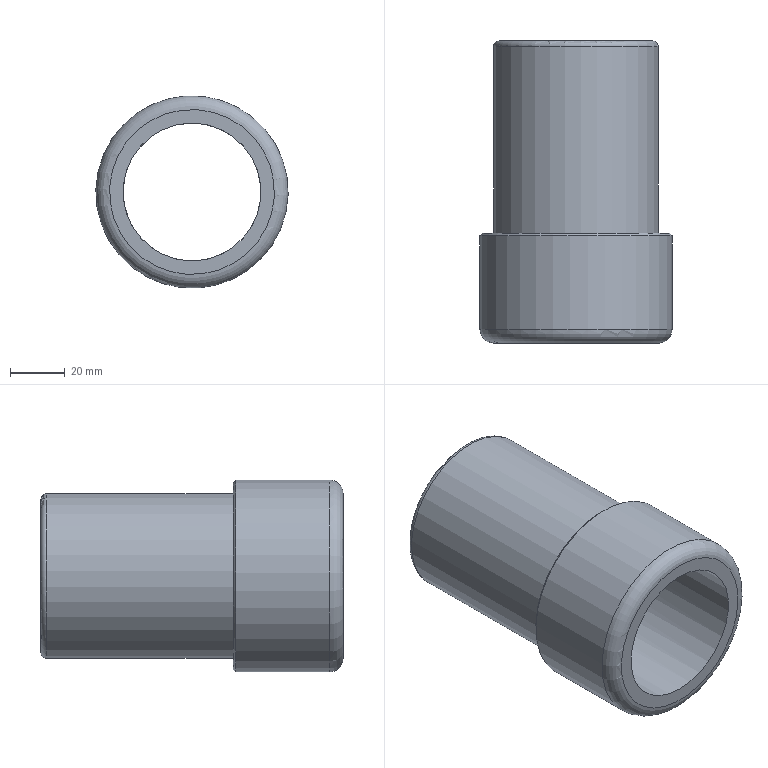Component | NX | BUSH | 1 solid | 10 faces | box 70 x 110 x 70 mm | volume 133028 mm3 | plane 3 | cylinder 3 | torus 3 | cone 1 | commonest cylinder face diameters 70 x1 60 x1 50.15 x1
STEP:
#1=CARTESIAN_POINT('',(0.,0.,0.));
#2=DIRECTION('',(0.,0.,1.));
#3=DIRECTION('',(1.,0.,0.));
#4=AXIS2_PLACEMENT_3D('',#1,#2,#3);
#5=CARTESIAN_POINT('',(-145.981,270.,-222.846));
#6=VERTEX_POINT('',#5);
#7=CARTESIAN_POINT('',(-120.,270.,-207.846));
#8=DIRECTION('',(-0.,-1.,-0.));
#9=DIRECTION('',(-0.866,0.,-0.5));
#10=AXIS2_PLACEMENT_3D('',#7,#8,#9);
#11=CIRCLE('',#10,30.);
#12=CARTESIAN_POINT('',(-120.,270.,-207.846));
#13=DIRECTION('',(0.,1.,0.));
#14=DIRECTION('',(-0.866,0.,-0.5));
#15=AXIS2_PLACEMENT_3D('',#12,#13,#14);
#16=PLANE('',#15);
#17=CARTESIAN_POINT('',(30.,0.));
#18=CARTESIAN_POINT('',(30.,-51.962));
#19=CARTESIAN_POINT('',(-15.,-25.981));
#20=CARTESIAN_POINT('',(-60.,-0.));
#21=CARTESIAN_POINT('',(-15.,25.981));
#22=CARTESIAN_POINT('',(30.,51.962));
#23=CARTESIAN_POINT('',(30.,0.));
#24=(BOUNDED_CURVE()B_SPLINE_CURVE(2,(#17,#18,#19,#20,#21,#22,#23),.UNSPECIFIED.,.T.,.F.)B_SPLINE_CURVE_WITH_KNOTS((1,2,2,2,2,1),(-2.094,0.,2.094,4.189,6.283,8.378),.UNSPECIFIED.)CURVE()GEOMETRIC_REPRESENTATION_ITEM()RATIONAL_B_SPLINE_CURVE((1.,0.5,1.,0.5,1.,0.5,1.))REPRESENTATION_ITEM(''));
#25=(GEOMETRIC_REPRESENTATION_CONTEXT(2)PARAMETRIC_REPRESENTATION_CONTEXT()REPRESENTATION_CONTEXT('',''));
#26=DEFINITIONAL_REPRESENTATION('',(#24),#25);
#27=PCURVE('',#16,#26);
#28=CARTESIAN_POINT('',(-120.,275.,-207.846));
#29=DIRECTION('',(0.,1.,0.));
#30=DIRECTION('',(-0.866,0.,-0.5));
#31=AXIS2_PLACEMENT_3D('',#28,#29,#30);
#32=TOROIDAL_SURFACE('',#31,30.,5.);
#33=CARTESIAN_POINT('',(6.283,4.712));
#34=DIRECTION('',(-1.,0.));
#35=VECTOR('',#34,1.);
#36=LINE('',#33,#35);
#37=(GEOMETRIC_REPRESENTATION_CONTEXT(2)PARAMETRIC_REPRESENTATION_CONTEXT()REPRESENTATION_CONTEXT('',''));
#38=DEFINITIONAL_REPRESENTATION('',(#36),#37);
#39=PCURVE('',#32,#38);
#40=SURFACE_CURVE('',#11,(#27,#39),.PCURVE_S1.);
#41=EDGE_CURVE('',#6,#6,#40,.T.);
#42=ORIENTED_EDGE('',*,*,#41,.T.);
#43=EDGE_LOOP('',(#42));
#44=FACE_BOUND('',#43,.T.);
#45=CARTESIAN_POINT('',(-141.716,270.,-220.384));
#46=VERTEX_POINT('',#45);
#47=CARTESIAN_POINT('',(-98.284,270.,-195.309));
#48=VERTEX_POINT('',#47);
#49=CARTESIAN_POINT('',(-120.,270.,-207.846));
#50=DIRECTION('',(0.,1.,0.));
#51=DIRECTION('',(-0.866,0.,-0.5));
#52=AXIS2_PLACEMENT_3D('',#49,#50,#51);
#53=CIRCLE('',#52,25.075);
#54=CARTESIAN_POINT('',(0.,0.));
#55=DIRECTION('',(1.,0.));
#56=AXIS2_PLACEMENT_2D('',#54,#55);
#57=CIRCLE('',#56,25.075);
#58=(GEOMETRIC_REPRESENTATION_CONTEXT(2)PARAMETRIC_REPRESENTATION_CONTEXT()REPRESENTATION_CONTEXT('',''));
#59=DEFINITIONAL_REPRESENTATION('',(#57),#58);
#60=PCURVE('',#16,#59);
#61=CARTESIAN_POINT('',(-120.,380.,-207.846));
#62=DIRECTION('',(-0.,-1.,-0.));
#63=DIRECTION('',(0.866,-0.,0.5));
#64=AXIS2_PLACEMENT_3D('',#61,#62,#63);
#65=CYLINDRICAL_SURFACE('',#64,25.075);
#66=CARTESIAN_POINT('',(3.142,110.));
#67=DIRECTION('',(-1.,0.));
#68=VECTOR('',#67,1.);
#69=LINE('',#66,#68);
#70=(GEOMETRIC_REPRESENTATION_CONTEXT(2)PARAMETRIC_REPRESENTATION_CONTEXT()REPRESENTATION_CONTEXT('',''));
#71=DEFINITIONAL_REPRESENTATION('',(#69),#70);
#72=PCURVE('',#65,#71);
#73=SURFACE_CURVE('',#53,(#60,#72),.PCURVE_S1.);
#74=EDGE_CURVE('',#46,#48,#73,.T.);
#75=ORIENTED_EDGE('',*,*,#74,.T.);
#76=CARTESIAN_POINT('',(-120.,270.,-207.846));
#77=DIRECTION('',(0.,1.,0.));
#78=DIRECTION('',(-0.866,0.,-0.5));
#79=AXIS2_PLACEMENT_3D('',#76,#77,#78);
#80=CIRCLE('',#79,25.075);
#81=CARTESIAN_POINT('',(0.,0.));
#82=DIRECTION('',(1.,0.));
#83=AXIS2_PLACEMENT_2D('',#81,#82);
#84=CIRCLE('',#83,25.075);
#85=(GEOMETRIC_REPRESENTATION_CONTEXT(2)PARAMETRIC_REPRESENTATION_CONTEXT()REPRESENTATION_CONTEXT('',''));
#86=DEFINITIONAL_REPRESENTATION('',(#84),#85);
#87=PCURVE('',#16,#86);
#88=CARTESIAN_POINT('',(9.425,110.));
#89=DIRECTION('',(-1.,0.));
#90=VECTOR('',#89,1.);
#91=LINE('',#88,#90);
#92=(GEOMETRIC_REPRESENTATION_CONTEXT(2)PARAMETRIC_REPRESENTATION_CONTEXT()REPRESENTATION_CONTEXT('',''));
#93=DEFINITIONAL_REPRESENTATION('',(#91),#92);
#94=PCURVE('',#65,#93);
#95=SURFACE_CURVE('',#80,(#87,#94),.PCURVE_S1.);
#96=EDGE_CURVE('',#48,#46,#95,.T.);
#97=ORIENTED_EDGE('',*,*,#96,.T.);
#98=EDGE_LOOP('',(#75,#97));
#99=FACE_BOUND('',#98,.T.);
#100=ADVANCED_FACE('',(#44,#99),#16,.F.);
#101=CARTESIAN_POINT('',(-89.689,309.,-190.346));
#102=VERTEX_POINT('',#101);
#103=CARTESIAN_POINT('',(-150.311,309.,-225.346));
#104=VERTEX_POINT('',#103);
#105=CARTESIAN_POINT('',(-120.,309.,-207.846));
#106=DIRECTION('',(-0.,-1.,-0.));
#107=DIRECTION('',(0.866,-0.,0.5));
#108=AXIS2_PLACEMENT_3D('',#105,#106,#107);
#109=CIRCLE('',#108,35.);
#110=CARTESIAN_POINT('',(-120.,270.,-207.846));
#111=DIRECTION('',(0.,1.,0.));
#112=DIRECTION('',(-0.866,0.,-0.5));
#113=AXIS2_PLACEMENT_3D('',#110,#111,#112);
#114=CYLINDRICAL_SURFACE('',#113,35.);
#115=CARTESIAN_POINT('',(3.142,39.));
#116=DIRECTION('',(-1.,0.));
#117=VECTOR('',#116,1.);
#118=LINE('',#115,#117);
#119=(GEOMETRIC_REPRESENTATION_CONTEXT(2)PARAMETRIC_REPRESENTATION_CONTEXT()REPRESENTATION_CONTEXT('',''));
#120=DEFINITIONAL_REPRESENTATION('',(#118),#119);
#121=PCURVE('',#114,#120);
#122=CARTESIAN_POINT('',(-120.,310.,-207.846));
#123=DIRECTION('',(-0.,-1.,-0.));
#124=DIRECTION('',(0.866,-0.,0.5));
#125=AXIS2_PLACEMENT_3D('',#122,#123,#124);
#126=CONICAL_SURFACE('',#125,34.,0.7854);
#127=CARTESIAN_POINT('',(0.,1.));
#128=DIRECTION('',(1.,0.));
#129=VECTOR('',#128,1.);
#130=LINE('',#127,#129);
#131=(GEOMETRIC_REPRESENTATION_CONTEXT(2)PARAMETRIC_REPRESENTATION_CONTEXT()REPRESENTATION_CONTEXT('',''));
#132=DEFINITIONAL_REPRESENTATION('',(#130),#131);
#133=PCURVE('',#126,#132);
#134=SURFACE_CURVE('',#109,(#121,#133),.PCURVE_S1.);
#135=EDGE_CURVE('',#102,#104,#134,.T.);
#136=ORIENTED_EDGE('',*,*,#135,.T.);
#137=CARTESIAN_POINT('',(-150.311,275.,-225.346));
#138=VERTEX_POINT('',#137);
#139=CARTESIAN_POINT('',(-150.311,275.,-225.346));
#140=CARTESIAN_POINT('',(-150.311,309.,-225.346));
#141=B_SPLINE_CURVE_WITH_KNOTS('',1,(#139,#140),.UNSPECIFIED.,.F.,.F.,(2,2),(5.,39.),.PIECEWISE_BEZIER_KNOTS.);
#142=CARTESIAN_POINT('',(0.,0.));
#143=DIRECTION('',(0.,1.));
#144=VECTOR('',#143,1.);
#145=LINE('',#142,#144);
#146=(GEOMETRIC_REPRESENTATION_CONTEXT(2)PARAMETRIC_REPRESENTATION_CONTEXT()REPRESENTATION_CONTEXT('',''));
#147=DEFINITIONAL_REPRESENTATION('',(#145),#146);
#148=PCURVE('',#114,#147);
#149=CARTESIAN_POINT('',(6.283,0.));
#150=DIRECTION('',(0.,1.));
#151=VECTOR('',#150,1.);
#152=LINE('',#149,#151);
#153=(GEOMETRIC_REPRESENTATION_CONTEXT(2)PARAMETRIC_REPRESENTATION_CONTEXT()REPRESENTATION_CONTEXT('',''));
#154=DEFINITIONAL_REPRESENTATION('',(#152),#153);
#155=PCURVE('',#114,#154);
#156=SEAM_CURVE('',#141,(#148,#155),.PCURVE_S1.);
#157=EDGE_CURVE('',#138,#104,#156,.T.);
#158=ORIENTED_EDGE('',*,*,#157,.F.);
#159=CARTESIAN_POINT('',(-120.,275.,-207.846));
#160=DIRECTION('',(0.,1.,0.));
#161=DIRECTION('',(-0.866,0.,-0.5));
#162=AXIS2_PLACEMENT_3D('',#159,#160,#161);
#163=CIRCLE('',#162,35.);
#164=CARTESIAN_POINT('',(0.,5.));
#165=DIRECTION('',(1.,0.));
#166=VECTOR('',#165,1.);
#167=LINE('',#164,#166);
#168=(GEOMETRIC_REPRESENTATION_CONTEXT(2)PARAMETRIC_REPRESENTATION_CONTEXT()REPRESENTATION_CONTEXT('',''));
#169=DEFINITIONAL_REPRESENTATION('',(#167),#168);
#170=PCURVE('',#114,#169);
#171=CARTESIAN_POINT('',(0.,6.283));
#172=DIRECTION('',(1.,0.));
#173=VECTOR('',#172,1.);
#174=LINE('',#171,#173);
#175=(GEOMETRIC_REPRESENTATION_CONTEXT(2)PARAMETRIC_REPRESENTATION_CONTEXT()REPRESENTATION_CONTEXT('',''));
#176=DEFINITIONAL_REPRESENTATION('',(#174),#175);
#177=PCURVE('',#32,#176);
#178=SURFACE_CURVE('',#163,(#170,#177),.PCURVE_S1.);
#179=EDGE_CURVE('',#138,#138,#178,.T.);
#180=ORIENTED_EDGE('',*,*,#179,.T.);
#181=ORIENTED_EDGE('',*,*,#157,.T.);
#182=CARTESIAN_POINT('',(-120.,309.,-207.846));
#183=DIRECTION('',(-0.,-1.,-0.));
#184=DIRECTION('',(0.866,-0.,0.5));
#185=AXIS2_PLACEMENT_3D('',#182,#183,#184);
#186=CIRCLE('',#185,35.);
#187=CARTESIAN_POINT('',(9.425,39.));
#188=DIRECTION('',(-1.,0.));
#189=VECTOR('',#188,1.);
#190=LINE('',#187,#189);
#191=(GEOMETRIC_REPRESENTATION_CONTEXT(2)PARAMETRIC_REPRESENTATION_CONTEXT()REPRESENTATION_CONTEXT('',''));
#192=DEFINITIONAL_REPRESENTATION('',(#190),#191);
#193=PCURVE('',#114,#192);
#194=CARTESIAN_POINT('',(0.,1.));
#195=DIRECTION('',(1.,-0.));
#196=VECTOR('',#195,1.);
#197=LINE('',#194,#196);
#198=(GEOMETRIC_REPRESENTATION_CONTEXT(2)PARAMETRIC_REPRESENTATION_CONTEXT()REPRESENTATION_CONTEXT('',''));
#199=DEFINITIONAL_REPRESENTATION('',(#197),#198);
#200=PCURVE('',#126,#199);
#201=SURFACE_CURVE('',#186,(#193,#200),.PCURVE_S1.);
#202=EDGE_CURVE('',#104,#102,#201,.T.);
#203=ORIENTED_EDGE('',*,*,#202,.T.);
#204=EDGE_LOOP('',(#136,#158,#180,#181,#203));
#205=FACE_BOUND('',#204,.T.);
#206=ADVANCED_FACE('',(#205),#114,.T.);
#207=CARTESIAN_POINT('',(-90.555,310.,-190.846));
#208=VERTEX_POINT('',#207);
#209=CARTESIAN_POINT('',(-120.,310.,-207.846));
#210=DIRECTION('',(0.,1.,0.));
#211=DIRECTION('',(0.866,-0.,0.5));
#212=AXIS2_PLACEMENT_3D('',#209,#210,#211);
#213=CIRCLE('',#212,34.);
#214=CARTESIAN_POINT('',(-89.689,310.,-190.346));
#215=DIRECTION('',(-0.,-1.,-0.));
#216=DIRECTION('',(0.866,-0.,0.5));
#217=AXIS2_PLACEMENT_3D('',#214,#215,#216);
#218=PLANE('',#217);
#219=CARTESIAN_POINT('',(-1.,0.));
#220=CARTESIAN_POINT('',(-1.,-58.89));
#221=CARTESIAN_POINT('',(-52.,-29.445));
#222=CARTESIAN_POINT('',(-103.,0.));
#223=CARTESIAN_POINT('',(-52.,29.445));
#224=CARTESIAN_POINT('',(-1.,58.89));
#225=CARTESIAN_POINT('',(-1.,0.));
#226=(BOUNDED_CURVE()B_SPLINE_CURVE(2,(#219,#220,#221,#222,#223,#224,#225),.UNSPECIFIED.,.T.,.F.)B_SPLINE_CURVE_WITH_KNOTS((1,2,2,2,2,1),(-2.094,0.,2.094,4.189,6.283,8.378),.UNSPECIFIED.)CURVE()GEOMETRIC_REPRESENTATION_ITEM()RATIONAL_B_SPLINE_CURVE((1.,0.5,1.,0.5,1.,0.5,1.))REPRESENTATION_ITEM(''));
#227=(GEOMETRIC_REPRESENTATION_CONTEXT(2)PARAMETRIC_REPRESENTATION_CONTEXT()REPRESENTATION_CONTEXT('',''));
#228=DEFINITIONAL_REPRESENTATION('',(#226),#227);
#229=PCURVE('',#218,#228);
#230=CARTESIAN_POINT('',(6.283,-0.));
#231=DIRECTION('',(-1.,0.));
#232=VECTOR('',#231,1.);
#233=LINE('',#230,#232);
#234=(GEOMETRIC_REPRESENTATION_CONTEXT(2)PARAMETRIC_REPRESENTATION_CONTEXT()REPRESENTATION_CONTEXT('',''));
#235=DEFINITIONAL_REPRESENTATION('',(#233),#234);
#236=PCURVE('',#126,#235);
#237=SURFACE_CURVE('',#213,(#229,#236),.PCURVE_S1.);
#238=EDGE_CURVE('',#208,#208,#237,.T.);
#239=ORIENTED_EDGE('',*,*,#238,.T.);
#240=EDGE_LOOP('',(#239));
#241=FACE_BOUND('',#240,.T.);
#242=CARTESIAN_POINT('',(-145.981,310.,-222.846));
#243=VERTEX_POINT('',#242);
#244=CARTESIAN_POINT('',(-120.,310.,-207.846));
#245=DIRECTION('',(0.,1.,0.));
#246=DIRECTION('',(-0.866,0.,-0.5));
#247=AXIS2_PLACEMENT_3D('',#244,#245,#246);
#248=CIRCLE('',#247,30.);
#249=CARTESIAN_POINT('',(-65.,0.));
#250=CARTESIAN_POINT('',(-65.,51.962));
#251=CARTESIAN_POINT('',(-20.,25.981));
#252=CARTESIAN_POINT('',(25.,0.));
#253=CARTESIAN_POINT('',(-20.,-25.981));
#254=CARTESIAN_POINT('',(-65.,-51.962));
#255=CARTESIAN_POINT('',(-65.,0.));
#256=(BOUNDED_CURVE()B_SPLINE_CURVE(2,(#249,#250,#251,#252,#253,#254,#255),.UNSPECIFIED.,.T.,.F.)B_SPLINE_CURVE_WITH_KNOTS((1,2,2,2,2,1),(-2.094,0.,2.094,4.189,6.283,8.378),.UNSPECIFIED.)CURVE()GEOMETRIC_REPRESENTATION_ITEM()RATIONAL_B_SPLINE_CURVE((1.,0.5,1.,0.5,1.,0.5,1.))REPRESENTATION_ITEM(''));
#257=(GEOMETRIC_REPRESENTATION_CONTEXT(2)PARAMETRIC_REPRESENTATION_CONTEXT()REPRESENTATION_CONTEXT('',''));
#258=DEFINITIONAL_REPRESENTATION('',(#256),#257);
#259=PCURVE('',#218,#258);
#260=CARTESIAN_POINT('',(-120.,270.,-207.846));
#261=DIRECTION('',(0.,1.,0.));
#262=DIRECTION('',(-0.866,0.,-0.5));
#263=AXIS2_PLACEMENT_3D('',#260,#261,#262);
#264=CYLINDRICAL_SURFACE('',#263,30.);
#265=CARTESIAN_POINT('',(0.,40.));
#266=DIRECTION('',(1.,0.));
#267=VECTOR('',#266,1.);
#268=LINE('',#265,#267);
#269=(GEOMETRIC_REPRESENTATION_CONTEXT(2)PARAMETRIC_REPRESENTATION_CONTEXT()REPRESENTATION_CONTEXT('',''));
#270=DEFINITIONAL_REPRESENTATION('',(#268),#269);
#271=PCURVE('',#264,#270);
#272=SURFACE_CURVE('',#248,(#259,#271),.PCURVE_S1.);
#273=EDGE_CURVE('',#243,#243,#272,.T.);
#274=ORIENTED_EDGE('',*,*,#273,.F.);
#275=EDGE_LOOP('',(#274));
#276=FACE_BOUND('',#275,.T.);
#277=ADVANCED_FACE('',(#241,#276),#218,.F.);
#278=CARTESIAN_POINT('',(-94.019,378.,-192.846));
#279=VERTEX_POINT('',#278);
#280=CARTESIAN_POINT('',(-145.981,378.,-222.846));
#281=VERTEX_POINT('',#280);
#282=CARTESIAN_POINT('',(-120.,378.,-207.846));
#283=DIRECTION('',(-0.,-1.,-0.));
#284=DIRECTION('',(0.866,-0.,0.5));
#285=AXIS2_PLACEMENT_3D('',#282,#283,#284);
#286=CIRCLE('',#285,30.);
#287=CARTESIAN_POINT('',(3.142,108.));
#288=DIRECTION('',(-1.,0.));
#289=VECTOR('',#288,1.);
#290=LINE('',#287,#289);
#291=(GEOMETRIC_REPRESENTATION_CONTEXT(2)PARAMETRIC_REPRESENTATION_CONTEXT()REPRESENTATION_CONTEXT('',''));
#292=DEFINITIONAL_REPRESENTATION('',(#290),#291);
#293=PCURVE('',#264,#292);
#294=CARTESIAN_POINT('',(-120.,378.,-207.846));
#295=DIRECTION('',(-0.,-1.,-0.));
#296=DIRECTION('',(0.866,-0.,0.5));
#297=AXIS2_PLACEMENT_3D('',#294,#295,#296);
#298=TOROIDAL_SURFACE('',#297,28.,2.);
#299=CARTESIAN_POINT('',(0.,6.283));
#300=DIRECTION('',(1.,0.));
#301=VECTOR('',#300,1.);
#302=LINE('',#299,#301);
#303=(GEOMETRIC_REPRESENTATION_CONTEXT(2)PARAMETRIC_REPRESENTATION_CONTEXT()REPRESENTATION_CONTEXT('',''));
#304=DEFINITIONAL_REPRESENTATION('',(#302),#303);
#305=PCURVE('',#298,#304);
#306=SURFACE_CURVE('',#286,(#293,#305),.PCURVE_S1.);
#307=EDGE_CURVE('',#279,#281,#306,.T.);
#308=ORIENTED_EDGE('',*,*,#307,.T.);
#309=CARTESIAN_POINT('',(-145.981,310.,-222.846));
#310=CARTESIAN_POINT('',(-145.981,378.,-222.846));
#311=B_SPLINE_CURVE_WITH_KNOTS('',1,(#309,#310),.UNSPECIFIED.,.F.,.F.,(2,2),(40.,108.),.PIECEWISE_BEZIER_KNOTS.);
#312=CARTESIAN_POINT('',(0.,0.));
#313=DIRECTION('',(0.,1.));
#314=VECTOR('',#313,1.);
#315=LINE('',#312,#314);
#316=(GEOMETRIC_REPRESENTATION_CONTEXT(2)PARAMETRIC_REPRESENTATION_CONTEXT()REPRESENTATION_CONTEXT('',''));
#317=DEFINITIONAL_REPRESENTATION('',(#315),#316);
#318=PCURVE('',#264,#317);
#319=CARTESIAN_POINT('',(6.283,0.));
#320=DIRECTION('',(0.,1.));
#321=VECTOR('',#320,1.);
#322=LINE('',#319,#321);
#323=(GEOMETRIC_REPRESENTATION_CONTEXT(2)PARAMETRIC_REPRESENTATION_CONTEXT()REPRESENTATION_CONTEXT('',''));
#324=DEFINITIONAL_REPRESENTATION('',(#322),#323);
#325=PCURVE('',#264,#324);
#326=SEAM_CURVE('',#311,(#318,#325),.PCURVE_S1.);
#327=EDGE_CURVE('',#243,#281,#326,.T.);
#328=ORIENTED_EDGE('',*,*,#327,.F.);
#329=ORIENTED_EDGE('',*,*,#273,.T.);
#330=ORIENTED_EDGE('',*,*,#327,.T.);
#331=CARTESIAN_POINT('',(-120.,378.,-207.846));
#332=DIRECTION('',(-0.,-1.,-0.));
#333=DIRECTION('',(0.866,-0.,0.5));
#334=AXIS2_PLACEMENT_3D('',#331,#332,#333);
#335=CIRCLE('',#334,30.);
#336=CARTESIAN_POINT('',(9.425,108.));
#337=DIRECTION('',(-1.,0.));
#338=VECTOR('',#337,1.);
#339=LINE('',#336,#338);
#340=(GEOMETRIC_REPRESENTATION_CONTEXT(2)PARAMETRIC_REPRESENTATION_CONTEXT()REPRESENTATION_CONTEXT('',''));
#341=DEFINITIONAL_REPRESENTATION('',(#339),#340);
#342=PCURVE('',#264,#341);
#343=CARTESIAN_POINT('',(0.,6.283));
#344=DIRECTION('',(1.,0.));
#345=VECTOR('',#344,1.);
#346=LINE('',#343,#345);
#347=(GEOMETRIC_REPRESENTATION_CONTEXT(2)PARAMETRIC_REPRESENTATION_CONTEXT()REPRESENTATION_CONTEXT('',''));
#348=DEFINITIONAL_REPRESENTATION('',(#346),#347);
#349=PCURVE('',#298,#348);
#350=SURFACE_CURVE('',#335,(#342,#349),.PCURVE_S1.);
#351=EDGE_CURVE('',#281,#279,#350,.T.);
#352=ORIENTED_EDGE('',*,*,#351,.T.);
#353=EDGE_LOOP('',(#308,#328,#329,#330,#352));
#354=FACE_BOUND('',#353,.T.);
#355=ADVANCED_FACE('',(#354),#264,.T.);
#356=CARTESIAN_POINT('',(-96.552,380.,-194.309));
#357=VERTEX_POINT('',#356);
#358=CARTESIAN_POINT('',(-120.,380.,-207.846));
#359=DIRECTION('',(-0.,-1.,-0.));
#360=DIRECTION('',(0.866,-0.,0.5));
#361=AXIS2_PLACEMENT_3D('',#358,#359,#360);
#362=CIRCLE('',#361,27.075);
#363=CARTESIAN_POINT('',(-94.019,380.,-192.846));
#364=DIRECTION('',(-0.,-1.,-0.));
#365=DIRECTION('',(0.866,-0.,0.5));
#366=AXIS2_PLACEMENT_3D('',#363,#364,#365);
#367=PLANE('',#366);
#368=CARTESIAN_POINT('',(-30.,0.));
#369=DIRECTION('',(1.,0.));
#370=AXIS2_PLACEMENT_2D('',#368,#369);
#371=CIRCLE('',#370,27.075);
#372=(GEOMETRIC_REPRESENTATION_CONTEXT(2)PARAMETRIC_REPRESENTATION_CONTEXT()REPRESENTATION_CONTEXT('',''));
#373=DEFINITIONAL_REPRESENTATION('',(#371),#372);
#374=PCURVE('',#367,#373);
#375=CARTESIAN_POINT('',(-120.,378.,-207.846));
#376=DIRECTION('',(-0.,-1.,-0.));
#377=DIRECTION('',(0.866,-0.,0.5));
#378=AXIS2_PLACEMENT_3D('',#375,#376,#377);
#379=TOROIDAL_SURFACE('',#378,27.075,2.);
#380=CARTESIAN_POINT('',(0.,4.712));
#381=DIRECTION('',(1.,0.));
#382=VECTOR('',#381,1.);
#383=LINE('',#380,#382);
#384=(GEOMETRIC_REPRESENTATION_CONTEXT(2)PARAMETRIC_REPRESENTATION_CONTEXT()REPRESENTATION_CONTEXT('',''));
#385=DEFINITIONAL_REPRESENTATION('',(#383),#384);
#386=PCURVE('',#379,#385);
#387=SURFACE_CURVE('',#362,(#374,#386),.PCURVE_S1.);
#388=EDGE_CURVE('',#357,#357,#387,.T.);
#389=ORIENTED_EDGE('',*,*,#388,.T.);
#390=EDGE_LOOP('',(#389));
#391=FACE_BOUND('',#390,.T.);
#392=CARTESIAN_POINT('',(-95.751,380.,-193.846));
#393=VERTEX_POINT('',#392);
#394=CARTESIAN_POINT('',(-120.,380.,-207.846));
#395=DIRECTION('',(0.,1.,0.));
#396=DIRECTION('',(0.866,-0.,0.5));
#397=AXIS2_PLACEMENT_3D('',#394,#395,#396);
#398=CIRCLE('',#397,28.);
#399=CARTESIAN_POINT('',(-2.,0.));
#400=CARTESIAN_POINT('',(-2.,-48.497));
#401=CARTESIAN_POINT('',(-44.,-24.249));
#402=CARTESIAN_POINT('',(-86.,0.));
#403=CARTESIAN_POINT('',(-44.,24.249));
#404=CARTESIAN_POINT('',(-2.,48.497));
#405=CARTESIAN_POINT('',(-2.,0.));
#406=(BOUNDED_CURVE()B_SPLINE_CURVE(2,(#399,#400,#401,#402,#403,#404,#405),.UNSPECIFIED.,.T.,.F.)B_SPLINE_CURVE_WITH_KNOTS((1,2,2,2,2,1),(-2.094,0.,2.094,4.189,6.283,8.378),.UNSPECIFIED.)CURVE()GEOMETRIC_REPRESENTATION_ITEM()RATIONAL_B_SPLINE_CURVE((1.,0.5,1.,0.5,1.,0.5,1.))REPRESENTATION_ITEM(''));
#407=(GEOMETRIC_REPRESENTATION_CONTEXT(2)PARAMETRIC_REPRESENTATION_CONTEXT()REPRESENTATION_CONTEXT('',''));
#408=DEFINITIONAL_REPRESENTATION('',(#406),#407);
#409=PCURVE('',#367,#408);
#410=CARTESIAN_POINT('',(6.283,4.712));
#411=DIRECTION('',(-1.,0.));
#412=VECTOR('',#411,1.);
#413=LINE('',#410,#412);
#414=(GEOMETRIC_REPRESENTATION_CONTEXT(2)PARAMETRIC_REPRESENTATION_CONTEXT()REPRESENTATION_CONTEXT('',''));
#415=DEFINITIONAL_REPRESENTATION('',(#413),#414);
#416=PCURVE('',#298,#415);
#417=SURFACE_CURVE('',#398,(#409,#416),.PCURVE_S1.);
#418=EDGE_CURVE('',#393,#393,#417,.T.);
#419=ORIENTED_EDGE('',*,*,#418,.T.);
#420=EDGE_LOOP('',(#419));
#421=FACE_BOUND('',#420,.T.);
#422=ADVANCED_FACE('',(#391,#421),#367,.F.);
#423=CARTESIAN_POINT('',(-98.284,378.,-195.309));
#424=VERTEX_POINT('',#423);
#425=CARTESIAN_POINT('',(-120.,378.,-207.846));
#426=DIRECTION('',(0.,1.,0.));
#427=DIRECTION('',(0.866,-0.,0.5));
#428=AXIS2_PLACEMENT_3D('',#425,#426,#427);
#429=CIRCLE('',#428,25.075);
#430=CARTESIAN_POINT('',(6.283,2.));
#431=DIRECTION('',(-1.,0.));
#432=VECTOR('',#431,1.);
#433=LINE('',#430,#432);
#434=(GEOMETRIC_REPRESENTATION_CONTEXT(2)PARAMETRIC_REPRESENTATION_CONTEXT()REPRESENTATION_CONTEXT('',''));
#435=DEFINITIONAL_REPRESENTATION('',(#433),#434);
#436=PCURVE('',#65,#435);
#437=CARTESIAN_POINT('',(6.283,3.142));
#438=DIRECTION('',(-1.,0.));
#439=VECTOR('',#438,1.);
#440=LINE('',#437,#439);
#441=(GEOMETRIC_REPRESENTATION_CONTEXT(2)PARAMETRIC_REPRESENTATION_CONTEXT()REPRESENTATION_CONTEXT('',''));
#442=DEFINITIONAL_REPRESENTATION('',(#440),#441);
#443=PCURVE('',#379,#442);
#444=SURFACE_CURVE('',#429,(#436,#443),.PCURVE_S1.);
#445=EDGE_CURVE('',#424,#424,#444,.T.);
#446=ORIENTED_EDGE('',*,*,#445,.F.);
#447=CARTESIAN_POINT('',(-98.284,378.,-195.309));
#448=CARTESIAN_POINT('',(-98.284,270.,-195.309));
#449=B_SPLINE_CURVE_WITH_KNOTS('',1,(#447,#448),.UNSPECIFIED.,.F.,.F.,(2,2),(2.,110.),.PIECEWISE_BEZIER_KNOTS.);
#450=CARTESIAN_POINT('',(6.283,0.));
#451=DIRECTION('',(0.,1.));
#452=VECTOR('',#451,1.);
#453=LINE('',#450,#452);
#454=(GEOMETRIC_REPRESENTATION_CONTEXT(2)PARAMETRIC_REPRESENTATION_CONTEXT()REPRESENTATION_CONTEXT('',''));
#455=DEFINITIONAL_REPRESENTATION('',(#453),#454);
#456=PCURVE('',#65,#455);
#457=CARTESIAN_POINT('',(0.,0.));
#458=DIRECTION('',(0.,1.));
#459=VECTOR('',#458,1.);
#460=LINE('',#457,#459);
#461=(GEOMETRIC_REPRESENTATION_CONTEXT(2)PARAMETRIC_REPRESENTATION_CONTEXT()REPRESENTATION_CONTEXT('',''));
#462=DEFINITIONAL_REPRESENTATION('',(#460),#461);
#463=PCURVE('',#65,#462);
#464=SEAM_CURVE('',#449,(#456,#463),.PCURVE_S1.);
#465=EDGE_CURVE('',#424,#48,#464,.T.);
#466=ORIENTED_EDGE('',*,*,#465,.T.);
#467=ORIENTED_EDGE('',*,*,#96,.T.);
#468=ORIENTED_EDGE('',*,*,#74,.T.);
#469=ORIENTED_EDGE('',*,*,#465,.F.);
#470=EDGE_LOOP('',(#446,#466,#467,#468,#469));
#471=FACE_BOUND('',#470,.F.);
#472=ADVANCED_FACE('',(#471),#65,.F.);
#473=ORIENTED_EDGE('',*,*,#41,.F.);
#474=CARTESIAN_POINT('',(-145.981,270.,-222.846));
#475=CARTESIAN_POINT('',(-147.138,270.,-223.514));
#476=CARTESIAN_POINT('',(-148.266,270.425,-224.165));
#477=CARTESIAN_POINT('',(-149.237,271.24,-224.726));
#478=CARTESIAN_POINT('',(-149.943,272.361,-225.134));
#479=CARTESIAN_POINT('',(-150.311,273.663,-225.346));
#480=CARTESIAN_POINT('',(-150.311,275.,-225.346));
#481=(BOUNDED_CURVE()B_SPLINE_CURVE(6,(#474,#475,#476,#477,#478,#479,#480),.UNSPECIFIED.,.F.,.F.)B_SPLINE_CURVE_WITH_KNOTS((7,7),(4.712,6.283),.PIECEWISE_BEZIER_KNOTS.)CURVE()GEOMETRIC_REPRESENTATION_ITEM()RATIONAL_B_SPLINE_CURVE((1.031,1.01,0.9979,0.994,0.9979,1.01,1.031))REPRESENTATION_ITEM(''));
#482=CARTESIAN_POINT('',(6.283,0.));
#483=DIRECTION('',(0.,1.));
#484=VECTOR('',#483,1.);
#485=LINE('',#482,#484);
#486=(GEOMETRIC_REPRESENTATION_CONTEXT(2)PARAMETRIC_REPRESENTATION_CONTEXT()REPRESENTATION_CONTEXT('',''));
#487=DEFINITIONAL_REPRESENTATION('',(#485),#486);
#488=PCURVE('',#32,#487);
#489=CARTESIAN_POINT('',(0.,0.));
#490=DIRECTION('',(0.,1.));
#491=VECTOR('',#490,1.);
#492=LINE('',#489,#491);
#493=(GEOMETRIC_REPRESENTATION_CONTEXT(2)PARAMETRIC_REPRESENTATION_CONTEXT()REPRESENTATION_CONTEXT('',''));
#494=DEFINITIONAL_REPRESENTATION('',(#492),#493);
#495=PCURVE('',#32,#494);
#496=SEAM_CURVE('',#481,(#488,#495),.PCURVE_S1.);
#497=EDGE_CURVE('',#6,#138,#496,.T.);
#498=ORIENTED_EDGE('',*,*,#497,.T.);
#499=ORIENTED_EDGE('',*,*,#179,.F.);
#500=ORIENTED_EDGE('',*,*,#497,.F.);
#501=EDGE_LOOP('',(#473,#498,#499,#500));
#502=FACE_BOUND('',#501,.T.);
#503=ADVANCED_FACE('',(#502),#32,.T.);
#504=ORIENTED_EDGE('',*,*,#445,.F.);
#505=CARTESIAN_POINT('',(-98.284,378.,-195.309));
#506=CARTESIAN_POINT('',(-98.284,378.535,-195.309));
#507=CARTESIAN_POINT('',(-98.137,379.055,-195.224));
#508=CARTESIAN_POINT('',(-97.855,379.504,-195.061));
#509=CARTESIAN_POINT('',(-97.466,379.83,-194.836));
#510=CARTESIAN_POINT('',(-97.015,380.,-194.576));
#511=CARTESIAN_POINT('',(-96.552,380.,-194.309));
#512=(BOUNDED_CURVE()B_SPLINE_CURVE(6,(#505,#506,#507,#508,#509,#510,#511),.UNSPECIFIED.,.F.,.F.)B_SPLINE_CURVE_WITH_KNOTS((7,7),(3.142,4.712),.PIECEWISE_BEZIER_KNOTS.)CURVE()GEOMETRIC_REPRESENTATION_ITEM()RATIONAL_B_SPLINE_CURVE((1.031,1.01,0.9979,0.994,0.9979,1.01,1.031))REPRESENTATION_ITEM(''));
#513=CARTESIAN_POINT('',(6.283,0.));
#514=DIRECTION('',(0.,1.));
#515=VECTOR('',#514,1.);
#516=LINE('',#513,#515);
#517=(GEOMETRIC_REPRESENTATION_CONTEXT(2)PARAMETRIC_REPRESENTATION_CONTEXT()REPRESENTATION_CONTEXT('',''));
#518=DEFINITIONAL_REPRESENTATION('',(#516),#517);
#519=PCURVE('',#379,#518);
#520=CARTESIAN_POINT('',(0.,0.));
#521=DIRECTION('',(0.,1.));
#522=VECTOR('',#521,1.);
#523=LINE('',#520,#522);
#524=(GEOMETRIC_REPRESENTATION_CONTEXT(2)PARAMETRIC_REPRESENTATION_CONTEXT()REPRESENTATION_CONTEXT('',''));
#525=DEFINITIONAL_REPRESENTATION('',(#523),#524);
#526=PCURVE('',#379,#525);
#527=SEAM_CURVE('',#512,(#519,#526),.PCURVE_S1.);
#528=EDGE_CURVE('',#424,#357,#527,.T.);
#529=ORIENTED_EDGE('',*,*,#528,.T.);
#530=ORIENTED_EDGE('',*,*,#388,.F.);
#531=ORIENTED_EDGE('',*,*,#528,.F.);
#532=EDGE_LOOP('',(#504,#529,#530,#531));
#533=FACE_BOUND('',#532,.T.);
#534=ADVANCED_FACE('',(#533),#379,.T.);
#535=ORIENTED_EDGE('',*,*,#307,.F.);
#536=CARTESIAN_POINT('',(-95.751,380.,-193.846));
#537=CARTESIAN_POINT('',(-95.288,380.,-193.579));
#538=CARTESIAN_POINT('',(-94.837,379.83,-193.318));
#539=CARTESIAN_POINT('',(-94.449,379.504,-193.094));
#540=CARTESIAN_POINT('',(-94.166,379.055,-192.931));
#541=CARTESIAN_POINT('',(-94.019,378.535,-192.846));
#542=CARTESIAN_POINT('',(-94.019,378.,-192.846));
#543=(BOUNDED_CURVE()B_SPLINE_CURVE(6,(#536,#537,#538,#539,#540,#541,#542),.UNSPECIFIED.,.F.,.F.)B_SPLINE_CURVE_WITH_KNOTS((7,7),(-1.571,0.),.PIECEWISE_BEZIER_KNOTS.)CURVE()GEOMETRIC_REPRESENTATION_ITEM()RATIONAL_B_SPLINE_CURVE((1.031,1.01,0.9979,0.994,0.9979,1.01,1.031))REPRESENTATION_ITEM(''));
#544=CARTESIAN_POINT('',(0.,6.283));
#545=DIRECTION('',(0.,1.));
#546=VECTOR('',#545,1.);
#547=LINE('',#544,#546);
#548=(GEOMETRIC_REPRESENTATION_CONTEXT(2)PARAMETRIC_REPRESENTATION_CONTEXT()REPRESENTATION_CONTEXT('',''));
#549=DEFINITIONAL_REPRESENTATION('',(#547),#548);
#550=PCURVE('',#298,#549);
#551=CARTESIAN_POINT('',(6.283,6.283));
#552=DIRECTION('',(0.,1.));
#553=VECTOR('',#552,1.);
#554=LINE('',#551,#553);
#555=(GEOMETRIC_REPRESENTATION_CONTEXT(2)PARAMETRIC_REPRESENTATION_CONTEXT()REPRESENTATION_CONTEXT('',''));
#556=DEFINITIONAL_REPRESENTATION('',(#554),#555);
#557=PCURVE('',#298,#556);
#558=SEAM_CURVE('',#543,(#550,#557),.PCURVE_S1.);
#559=EDGE_CURVE('',#393,#279,#558,.T.);
#560=ORIENTED_EDGE('',*,*,#559,.F.);
#561=ORIENTED_EDGE('',*,*,#418,.F.);
#562=ORIENTED_EDGE('',*,*,#559,.T.);
#563=ORIENTED_EDGE('',*,*,#351,.F.);
#564=EDGE_LOOP('',(#535,#560,#561,#562,#563));
#565=FACE_BOUND('',#564,.T.);
#566=ADVANCED_FACE('',(#565),#298,.T.);
#567=ORIENTED_EDGE('',*,*,#135,.F.);
#568=CARTESIAN_POINT('',(-90.555,310.,-190.846));
#569=CARTESIAN_POINT('',(-89.689,309.,-190.346));
#570=B_SPLINE_CURVE_WITH_KNOTS('',1,(#568,#569),.UNSPECIFIED.,.F.,.F.,(2,2),(-0.,1.414),.PIECEWISE_BEZIER_KNOTS.);
#571=CARTESIAN_POINT('',(0.,0.));
#572=DIRECTION('',(0.,1.));
#573=VECTOR('',#572,1.);
#574=LINE('',#571,#573);
#575=(GEOMETRIC_REPRESENTATION_CONTEXT(2)PARAMETRIC_REPRESENTATION_CONTEXT()REPRESENTATION_CONTEXT('',''));
#576=DEFINITIONAL_REPRESENTATION('',(#574),#575);
#577=PCURVE('',#126,#576);
#578=CARTESIAN_POINT('',(6.283,0.));
#579=DIRECTION('',(0.,1.));
#580=VECTOR('',#579,1.);
#581=LINE('',#578,#580);
#582=(GEOMETRIC_REPRESENTATION_CONTEXT(2)PARAMETRIC_REPRESENTATION_CONTEXT()REPRESENTATION_CONTEXT('',''));
#583=DEFINITIONAL_REPRESENTATION('',(#581),#582);
#584=PCURVE('',#126,#583);
#585=SEAM_CURVE('',#570,(#577,#584),.PCURVE_S1.);
#586=EDGE_CURVE('',#208,#102,#585,.T.);
#587=ORIENTED_EDGE('',*,*,#586,.F.);
#588=ORIENTED_EDGE('',*,*,#238,.F.);
#589=ORIENTED_EDGE('',*,*,#586,.T.);
#590=ORIENTED_EDGE('',*,*,#202,.F.);
#591=EDGE_LOOP('',(#567,#587,#588,#589,#590));
#592=FACE_BOUND('',#591,.T.);
#593=ADVANCED_FACE('',(#592),#126,.T.);
#594=CLOSED_SHELL('',(#100,#206,#277,#355,#422,#472,#503,#534,#566,#593));
#595=MANIFOLD_SOLID_BREP('',#594);
#596=(LENGTH_UNIT()NAMED_UNIT(*)SI_UNIT(.MILLI.,.METRE.));
#597=UNCERTAINTY_MEASURE_WITH_UNIT(LENGTH_MEASURE(0.00001),#596,'','');
#598=(NAMED_UNIT(*)PLANE_ANGLE_UNIT()SI_UNIT($,.RADIAN.));
#599=(NAMED_UNIT(*)SI_UNIT($,.STERADIAN.)SOLID_ANGLE_UNIT());
#600=(GEOMETRIC_REPRESENTATION_CONTEXT(3)GLOBAL_UNCERTAINTY_ASSIGNED_CONTEXT((#597))GLOBAL_UNIT_ASSIGNED_CONTEXT((#596,#598,#599))REPRESENTATION_CONTEXT('',''));
#601=ADVANCED_BREP_SHAPE_REPRESENTATION('',(#4,#595),#600);